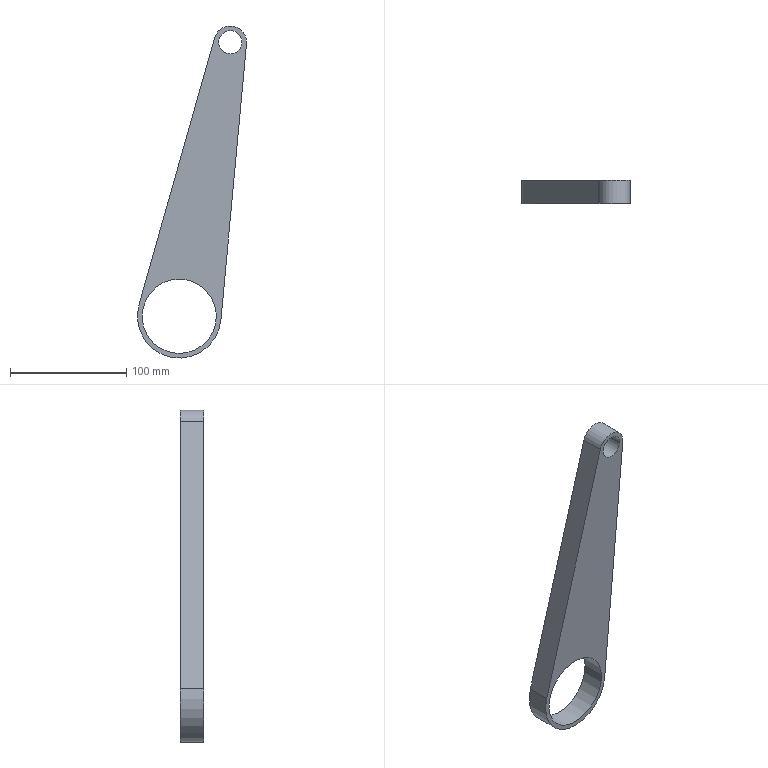Component | NX | CONNECTING_ROD | 1 solid | 8 faces | box 94 x 20 x 285.93 mm | volume 217259 mm3 | plane 4 | cylinder 4 | commonest cylinder face diameters 72 x1 64 x1 28 x1 20 x1
STEP:
#1=CARTESIAN_POINT('',(0.,0.,0.));
#2=DIRECTION('',(0.,0.,1.));
#3=DIRECTION('',(1.,0.,0.));
#4=AXIS2_PLACEMENT_3D('',#1,#2,#3);
#5=CARTESIAN_POINT('',(13.94,312.,234.638));
#6=VERTEX_POINT('',#5);
#7=CARTESIAN_POINT('',(-8.154,312.,-3.328));
#8=VERTEX_POINT('',#7);
#9=CARTESIAN_POINT('',(13.94,312.,234.638));
#10=DIRECTION('',(-0.09245,0.,-0.9957));
#11=VECTOR('',#10,1.);
#12=LINE('',#9,#11);
#13=CARTESIAN_POINT('',(13.94,292.,234.638));
#14=DIRECTION('',(0.9957,0.,-0.09245));
#15=DIRECTION('',(0.09245,0.,0.9957));
#16=AXIS2_PLACEMENT_3D('',#13,#14,#15);
#17=PLANE('',#16);
#18=CARTESIAN_POINT('',(0.,-20.));
#19=DIRECTION('',(-1.,0.));
#20=VECTOR('',#19,1.);
#21=LINE('',#18,#20);
#22=(GEOMETRIC_REPRESENTATION_CONTEXT(2)PARAMETRIC_REPRESENTATION_CONTEXT()REPRESENTATION_CONTEXT('',''));
#23=DEFINITIONAL_REPRESENTATION('',(#21),#22);
#24=PCURVE('',#17,#23);
#25=CARTESIAN_POINT('',(-44.,312.,0.));
#26=DIRECTION('',(0.,1.,0.));
#27=DIRECTION('',(-0.1833,0.,-0.9831));
#28=AXIS2_PLACEMENT_3D('',#25,#26,#27);
#29=PLANE('',#28);
#30=CARTESIAN_POINT('',(-241.283,-13.941));
#31=DIRECTION('',(0.9958,-0.09167));
#32=VECTOR('',#31,1.);
#33=LINE('',#30,#32);
#34=(GEOMETRIC_REPRESENTATION_CONTEXT(2)PARAMETRIC_REPRESENTATION_CONTEXT()REPRESENTATION_CONTEXT('',''));
#35=DEFINITIONAL_REPRESENTATION('',(#33),#34);
#36=PCURVE('',#29,#35);
#37=SURFACE_CURVE('',#12,(#24,#36),.PCURVE_S1.);
#38=EDGE_CURVE('',#6,#8,#37,.T.);
#39=ORIENTED_EDGE('',*,*,#38,.F.);
#40=CARTESIAN_POINT('',(13.94,292.,234.638));
#41=VERTEX_POINT('',#40);
#42=CARTESIAN_POINT('',(13.94,292.,234.638));
#43=DIRECTION('',(0.,1.,0.));
#44=VECTOR('',#43,1.);
#45=LINE('',#42,#44);
#46=CARTESIAN_POINT('',(0.,0.));
#47=DIRECTION('',(0.,-1.));
#48=VECTOR('',#47,1.);
#49=LINE('',#46,#48);
#50=(GEOMETRIC_REPRESENTATION_CONTEXT(2)PARAMETRIC_REPRESENTATION_CONTEXT()REPRESENTATION_CONTEXT('',''));
#51=DEFINITIONAL_REPRESENTATION('',(#49),#50);
#52=PCURVE('',#17,#51);
#53=CARTESIAN_POINT('',(0.,292.,235.932));
#54=DIRECTION('',(0.,1.,0.));
#55=DIRECTION('',(-0.1833,0.,-0.9831));
#56=AXIS2_PLACEMENT_3D('',#53,#54,#55);
#57=CYLINDRICAL_SURFACE('',#56,14.);
#58=CARTESIAN_POINT('',(4.621,0.));
#59=DIRECTION('',(0.,1.));
#60=VECTOR('',#59,1.);
#61=LINE('',#58,#60);
#62=(GEOMETRIC_REPRESENTATION_CONTEXT(2)PARAMETRIC_REPRESENTATION_CONTEXT()REPRESENTATION_CONTEXT('',''));
#63=DEFINITIONAL_REPRESENTATION('',(#61),#62);
#64=PCURVE('',#57,#63);
#65=SURFACE_CURVE('',#45,(#52,#64),.PCURVE_S1.);
#66=EDGE_CURVE('',#41,#6,#65,.T.);
#67=ORIENTED_EDGE('',*,*,#66,.F.);
#68=CARTESIAN_POINT('',(-8.154,292.,-3.328));
#69=VERTEX_POINT('',#68);
#70=CARTESIAN_POINT('',(13.94,292.,234.638));
#71=DIRECTION('',(-0.09245,0.,-0.9957));
#72=VECTOR('',#71,1.);
#73=LINE('',#70,#72);
#74=CARTESIAN_POINT('',(0.,0.));
#75=DIRECTION('',(-1.,0.));
#76=VECTOR('',#75,1.);
#77=LINE('',#74,#76);
#78=(GEOMETRIC_REPRESENTATION_CONTEXT(2)PARAMETRIC_REPRESENTATION_CONTEXT()REPRESENTATION_CONTEXT('',''));
#79=DEFINITIONAL_REPRESENTATION('',(#77),#78);
#80=PCURVE('',#17,#79);
#81=CARTESIAN_POINT('',(-44.,292.,0.));
#82=DIRECTION('',(0.,1.,0.));
#83=DIRECTION('',(-0.1833,0.,-0.9831));
#84=AXIS2_PLACEMENT_3D('',#81,#82,#83);
#85=PLANE('',#84);
#86=CARTESIAN_POINT('',(-241.283,-13.941));
#87=DIRECTION('',(0.9958,-0.09167));
#88=VECTOR('',#87,1.);
#89=LINE('',#86,#88);
#90=(GEOMETRIC_REPRESENTATION_CONTEXT(2)PARAMETRIC_REPRESENTATION_CONTEXT()REPRESENTATION_CONTEXT('',''));
#91=DEFINITIONAL_REPRESENTATION('',(#89),#90);
#92=PCURVE('',#85,#91);
#93=SURFACE_CURVE('',#73,(#80,#92),.PCURVE_S1.);
#94=EDGE_CURVE('',#41,#69,#93,.T.);
#95=ORIENTED_EDGE('',*,*,#94,.T.);
#96=CARTESIAN_POINT('',(-8.154,292.,-3.328));
#97=DIRECTION('',(0.,1.,0.));
#98=VECTOR('',#97,1.);
#99=LINE('',#96,#98);
#100=CARTESIAN_POINT('',(-238.99,0.));
#101=DIRECTION('',(0.,-1.));
#102=VECTOR('',#101,1.);
#103=LINE('',#100,#102);
#104=(GEOMETRIC_REPRESENTATION_CONTEXT(2)PARAMETRIC_REPRESENTATION_CONTEXT()REPRESENTATION_CONTEXT('',''));
#105=DEFINITIONAL_REPRESENTATION('',(#103),#104);
#106=PCURVE('',#17,#105);
#107=CARTESIAN_POINT('',(-44.,292.,0.));
#108=DIRECTION('',(0.,1.,0.));
#109=DIRECTION('',(-0.1833,0.,-0.9831));
#110=AXIS2_PLACEMENT_3D('',#107,#108,#109);
#111=CYLINDRICAL_SURFACE('',#110,36.);
#112=CARTESIAN_POINT('',(4.621,0.));
#113=DIRECTION('',(0.,1.));
#114=VECTOR('',#113,1.);
#115=LINE('',#112,#114);
#116=(GEOMETRIC_REPRESENTATION_CONTEXT(2)PARAMETRIC_REPRESENTATION_CONTEXT()REPRESENTATION_CONTEXT('',''));
#117=DEFINITIONAL_REPRESENTATION('',(#115),#116);
#118=PCURVE('',#111,#117);
#119=SURFACE_CURVE('',#99,(#106,#118),.PCURVE_S1.);
#120=EDGE_CURVE('',#69,#8,#119,.T.);
#121=ORIENTED_EDGE('',*,*,#120,.T.);
#122=EDGE_LOOP('',(#39,#67,#95,#121));
#123=FACE_BOUND('',#122,.T.);
#124=ADVANCED_FACE('',(#123),#17,.T.);
#125=CARTESIAN_POINT('',(-78.636,312.,9.816));
#126=VERTEX_POINT('',#125);
#127=CARTESIAN_POINT('',(-44.,312.,0.));
#128=DIRECTION('',(0.,1.,0.));
#129=DIRECTION('',(-0.9831,0.,0.1833));
#130=AXIS2_PLACEMENT_3D('',#127,#128,#129);
#131=CIRCLE('',#130,36.);
#132=CARTESIAN_POINT('',(1.571,20.));
#133=DIRECTION('',(1.,0.));
#134=VECTOR('',#133,1.);
#135=LINE('',#132,#134);
#136=(GEOMETRIC_REPRESENTATION_CONTEXT(2)PARAMETRIC_REPRESENTATION_CONTEXT()REPRESENTATION_CONTEXT('',''));
#137=DEFINITIONAL_REPRESENTATION('',(#135),#136);
#138=PCURVE('',#111,#137);
#139=CARTESIAN_POINT('',(0.,0.));
#140=DIRECTION('',(0.,1.));
#141=AXIS2_PLACEMENT_2D('',#139,#140);
#142=CIRCLE('',#141,36.);
#143=(GEOMETRIC_REPRESENTATION_CONTEXT(2)PARAMETRIC_REPRESENTATION_CONTEXT()REPRESENTATION_CONTEXT('',''));
#144=DEFINITIONAL_REPRESENTATION('',(#142),#143);
#145=PCURVE('',#29,#144);
#146=SURFACE_CURVE('',#131,(#138,#145),.PCURVE_S1.);
#147=EDGE_CURVE('',#8,#126,#146,.T.);
#148=ORIENTED_EDGE('',*,*,#147,.F.);
#149=ORIENTED_EDGE('',*,*,#120,.F.);
#150=CARTESIAN_POINT('',(-78.636,292.,9.816));
#151=VERTEX_POINT('',#150);
#152=CARTESIAN_POINT('',(-44.,292.,0.));
#153=DIRECTION('',(0.,1.,0.));
#154=DIRECTION('',(-0.9831,0.,0.1833));
#155=AXIS2_PLACEMENT_3D('',#152,#153,#154);
#156=CIRCLE('',#155,36.);
#157=CARTESIAN_POINT('',(1.571,0.));
#158=DIRECTION('',(1.,0.));
#159=VECTOR('',#158,1.);
#160=LINE('',#157,#159);
#161=(GEOMETRIC_REPRESENTATION_CONTEXT(2)PARAMETRIC_REPRESENTATION_CONTEXT()REPRESENTATION_CONTEXT('',''));
#162=DEFINITIONAL_REPRESENTATION('',(#160),#161);
#163=PCURVE('',#111,#162);
#164=CARTESIAN_POINT('',(0.,0.));
#165=DIRECTION('',(0.,1.));
#166=AXIS2_PLACEMENT_2D('',#164,#165);
#167=CIRCLE('',#166,36.);
#168=(GEOMETRIC_REPRESENTATION_CONTEXT(2)PARAMETRIC_REPRESENTATION_CONTEXT()REPRESENTATION_CONTEXT('',''));
#169=DEFINITIONAL_REPRESENTATION('',(#167),#168);
#170=PCURVE('',#85,#169);
#171=SURFACE_CURVE('',#156,(#163,#170),.PCURVE_S1.);
#172=EDGE_CURVE('',#69,#151,#171,.T.);
#173=ORIENTED_EDGE('',*,*,#172,.T.);
#174=CARTESIAN_POINT('',(-78.636,292.,9.816));
#175=DIRECTION('',(0.,1.,0.));
#176=VECTOR('',#175,1.);
#177=LINE('',#174,#176);
#178=CARTESIAN_POINT('',(7.946,0.));
#179=DIRECTION('',(0.,1.));
#180=VECTOR('',#179,1.);
#181=LINE('',#178,#180);
#182=(GEOMETRIC_REPRESENTATION_CONTEXT(2)PARAMETRIC_REPRESENTATION_CONTEXT()REPRESENTATION_CONTEXT('',''));
#183=DEFINITIONAL_REPRESENTATION('',(#181),#182);
#184=PCURVE('',#111,#183);
#185=CARTESIAN_POINT('',(-78.636,292.,9.816));
#186=DIRECTION('',(-0.9621,0.,0.2727));
#187=DIRECTION('',(-0.2727,0.,-0.9621));
#188=AXIS2_PLACEMENT_3D('',#185,#186,#187);
#189=PLANE('',#188);
#190=CARTESIAN_POINT('',(0.,0.));
#191=DIRECTION('',(0.,-1.));
#192=VECTOR('',#191,1.);
#193=LINE('',#190,#192);
#194=(GEOMETRIC_REPRESENTATION_CONTEXT(2)PARAMETRIC_REPRESENTATION_CONTEXT()REPRESENTATION_CONTEXT('',''));
#195=DEFINITIONAL_REPRESENTATION('',(#193),#194);
#196=PCURVE('',#189,#195);
#197=SURFACE_CURVE('',#177,(#184,#196),.PCURVE_S1.);
#198=EDGE_CURVE('',#151,#126,#197,.T.);
#199=ORIENTED_EDGE('',*,*,#198,.T.);
#200=EDGE_LOOP('',(#148,#149,#173,#199));
#201=FACE_BOUND('',#200,.T.);
#202=ADVANCED_FACE('',(#201),#111,.T.);
#203=CARTESIAN_POINT('',(-13.469,312.,239.75));
#204=VERTEX_POINT('',#203);
#205=CARTESIAN_POINT('',(-78.636,312.,9.816));
#206=DIRECTION('',(0.2727,0.,0.9621));
#207=VECTOR('',#206,1.);
#208=LINE('',#205,#207);
#209=CARTESIAN_POINT('',(0.,-20.));
#210=DIRECTION('',(-1.,0.));
#211=VECTOR('',#210,1.);
#212=LINE('',#209,#211);
#213=(GEOMETRIC_REPRESENTATION_CONTEXT(2)PARAMETRIC_REPRESENTATION_CONTEXT()REPRESENTATION_CONTEXT('',''));
#214=DEFINITIONAL_REPRESENTATION('',(#212),#213);
#215=PCURVE('',#189,#214);
#216=CARTESIAN_POINT('',(-3.3,35.848));
#217=DIRECTION('',(-0.9958,-0.09167));
#218=VECTOR('',#217,1.);
#219=LINE('',#216,#218);
#220=(GEOMETRIC_REPRESENTATION_CONTEXT(2)PARAMETRIC_REPRESENTATION_CONTEXT()REPRESENTATION_CONTEXT('',''));
#221=DEFINITIONAL_REPRESENTATION('',(#219),#220);
#222=PCURVE('',#29,#221);
#223=SURFACE_CURVE('',#208,(#215,#222),.PCURVE_S1.);
#224=EDGE_CURVE('',#126,#204,#223,.T.);
#225=ORIENTED_EDGE('',*,*,#224,.F.);
#226=ORIENTED_EDGE('',*,*,#198,.F.);
#227=CARTESIAN_POINT('',(-13.469,292.,239.75));
#228=VERTEX_POINT('',#227);
#229=CARTESIAN_POINT('',(-78.636,292.,9.816));
#230=DIRECTION('',(0.2727,0.,0.9621));
#231=VECTOR('',#230,1.);
#232=LINE('',#229,#231);
#233=CARTESIAN_POINT('',(0.,0.));
#234=DIRECTION('',(-1.,0.));
#235=VECTOR('',#234,1.);
#236=LINE('',#233,#235);
#237=(GEOMETRIC_REPRESENTATION_CONTEXT(2)PARAMETRIC_REPRESENTATION_CONTEXT()REPRESENTATION_CONTEXT('',''));
#238=DEFINITIONAL_REPRESENTATION('',(#236),#237);
#239=PCURVE('',#189,#238);
#240=CARTESIAN_POINT('',(-3.3,35.848));
#241=DIRECTION('',(-0.9958,-0.09167));
#242=VECTOR('',#241,1.);
#243=LINE('',#240,#242);
#244=(GEOMETRIC_REPRESENTATION_CONTEXT(2)PARAMETRIC_REPRESENTATION_CONTEXT()REPRESENTATION_CONTEXT('',''));
#245=DEFINITIONAL_REPRESENTATION('',(#243),#244);
#246=PCURVE('',#85,#245);
#247=SURFACE_CURVE('',#232,(#239,#246),.PCURVE_S1.);
#248=EDGE_CURVE('',#151,#228,#247,.T.);
#249=ORIENTED_EDGE('',*,*,#248,.T.);
#250=CARTESIAN_POINT('',(-13.469,292.,239.75));
#251=DIRECTION('',(0.,1.,0.));
#252=VECTOR('',#251,1.);
#253=LINE('',#250,#252);
#254=CARTESIAN_POINT('',(-238.99,0.));
#255=DIRECTION('',(0.,-1.));
#256=VECTOR('',#255,1.);
#257=LINE('',#254,#256);
#258=(GEOMETRIC_REPRESENTATION_CONTEXT(2)PARAMETRIC_REPRESENTATION_CONTEXT()REPRESENTATION_CONTEXT('',''));
#259=DEFINITIONAL_REPRESENTATION('',(#257),#258);
#260=PCURVE('',#189,#259);
#261=CARTESIAN_POINT('',(1.663,0.));
#262=DIRECTION('',(0.,1.));
#263=VECTOR('',#262,1.);
#264=LINE('',#261,#263);
#265=(GEOMETRIC_REPRESENTATION_CONTEXT(2)PARAMETRIC_REPRESENTATION_CONTEXT()REPRESENTATION_CONTEXT('',''));
#266=DEFINITIONAL_REPRESENTATION('',(#264),#265);
#267=PCURVE('',#57,#266);
#268=SURFACE_CURVE('',#253,(#260,#267),.PCURVE_S1.);
#269=EDGE_CURVE('',#228,#204,#268,.T.);
#270=ORIENTED_EDGE('',*,*,#269,.T.);
#271=EDGE_LOOP('',(#225,#226,#249,#270));
#272=FACE_BOUND('',#271,.T.);
#273=ADVANCED_FACE('',(#272),#189,.T.);
#274=CARTESIAN_POINT('',(-75.458,292.,5.867));
#275=VERTEX_POINT('',#274);
#276=CARTESIAN_POINT('',(-44.,292.,0.));
#277=DIRECTION('',(0.,1.,0.));
#278=DIRECTION('',(-0.9831,0.,0.1833));
#279=AXIS2_PLACEMENT_3D('',#276,#277,#278);
#280=CIRCLE('',#279,32.);
#281=CARTESIAN_POINT('',(-44.,292.,0.));
#282=DIRECTION('',(0.,1.,0.));
#283=DIRECTION('',(-0.1833,0.,-0.9831));
#284=AXIS2_PLACEMENT_3D('',#281,#282,#283);
#285=CYLINDRICAL_SURFACE('',#284,32.);
#286=CARTESIAN_POINT('',(1.571,0.));
#287=DIRECTION('',(1.,0.));
#288=VECTOR('',#287,1.);
#289=LINE('',#286,#288);
#290=(GEOMETRIC_REPRESENTATION_CONTEXT(2)PARAMETRIC_REPRESENTATION_CONTEXT()REPRESENTATION_CONTEXT('',''));
#291=DEFINITIONAL_REPRESENTATION('',(#289),#290);
#292=PCURVE('',#285,#291);
#293=CARTESIAN_POINT('',(0.,0.));
#294=DIRECTION('',(0.,1.));
#295=AXIS2_PLACEMENT_2D('',#293,#294);
#296=CIRCLE('',#295,32.);
#297=(GEOMETRIC_REPRESENTATION_CONTEXT(2)PARAMETRIC_REPRESENTATION_CONTEXT()REPRESENTATION_CONTEXT('',''));
#298=DEFINITIONAL_REPRESENTATION('',(#296),#297);
#299=PCURVE('',#85,#298);
#300=SURFACE_CURVE('',#280,(#292,#299),.PCURVE_S1.);
#301=EDGE_CURVE('',#275,#275,#300,.T.);
#302=ORIENTED_EDGE('',*,*,#301,.T.);
#303=CARTESIAN_POINT('',(-75.458,312.,5.867));
#304=VERTEX_POINT('',#303);
#305=CARTESIAN_POINT('',(-75.458,292.,5.867));
#306=CARTESIAN_POINT('',(-75.458,312.,5.867));
#307=B_SPLINE_CURVE_WITH_KNOTS('',1,(#305,#306),.UNSPECIFIED.,.F.,.F.,(2,2),(0.,20.),.PIECEWISE_BEZIER_KNOTS.);
#308=CARTESIAN_POINT('',(7.854,0.));
#309=DIRECTION('',(0.,1.));
#310=VECTOR('',#309,1.);
#311=LINE('',#308,#310);
#312=(GEOMETRIC_REPRESENTATION_CONTEXT(2)PARAMETRIC_REPRESENTATION_CONTEXT()REPRESENTATION_CONTEXT('',''));
#313=DEFINITIONAL_REPRESENTATION('',(#311),#312);
#314=PCURVE('',#285,#313);
#315=CARTESIAN_POINT('',(1.571,0.));
#316=DIRECTION('',(0.,1.));
#317=VECTOR('',#316,1.);
#318=LINE('',#315,#317);
#319=(GEOMETRIC_REPRESENTATION_CONTEXT(2)PARAMETRIC_REPRESENTATION_CONTEXT()REPRESENTATION_CONTEXT('',''));
#320=DEFINITIONAL_REPRESENTATION('',(#318),#319);
#321=PCURVE('',#285,#320);
#322=SEAM_CURVE('',#307,(#314,#321),.PCURVE_S1.);
#323=EDGE_CURVE('',#275,#304,#322,.T.);
#324=ORIENTED_EDGE('',*,*,#323,.T.);
#325=CARTESIAN_POINT('',(-44.,312.,0.));
#326=DIRECTION('',(0.,1.,0.));
#327=DIRECTION('',(-0.9831,0.,0.1833));
#328=AXIS2_PLACEMENT_3D('',#325,#326,#327);
#329=CIRCLE('',#328,32.);
#330=CARTESIAN_POINT('',(1.571,20.));
#331=DIRECTION('',(1.,0.));
#332=VECTOR('',#331,1.);
#333=LINE('',#330,#332);
#334=(GEOMETRIC_REPRESENTATION_CONTEXT(2)PARAMETRIC_REPRESENTATION_CONTEXT()REPRESENTATION_CONTEXT('',''));
#335=DEFINITIONAL_REPRESENTATION('',(#333),#334);
#336=PCURVE('',#285,#335);
#337=CARTESIAN_POINT('',(0.,0.));
#338=DIRECTION('',(0.,1.));
#339=AXIS2_PLACEMENT_2D('',#337,#338);
#340=CIRCLE('',#339,32.);
#341=(GEOMETRIC_REPRESENTATION_CONTEXT(2)PARAMETRIC_REPRESENTATION_CONTEXT()REPRESENTATION_CONTEXT('',''));
#342=DEFINITIONAL_REPRESENTATION('',(#340),#341);
#343=PCURVE('',#29,#342);
#344=SURFACE_CURVE('',#329,(#336,#343),.PCURVE_S1.);
#345=EDGE_CURVE('',#304,#304,#344,.T.);
#346=ORIENTED_EDGE('',*,*,#345,.F.);
#347=ORIENTED_EDGE('',*,*,#323,.F.);
#348=EDGE_LOOP('',(#302,#324,#346,#347));
#349=FACE_BOUND('',#348,.F.);
#350=ADVANCED_FACE('',(#349),#285,.F.);
#351=CARTESIAN_POINT('',(0.,312.,235.932));
#352=DIRECTION('',(0.,1.,0.));
#353=DIRECTION('',(-0.9831,0.,0.1833));
#354=AXIS2_PLACEMENT_3D('',#351,#352,#353);
#355=CIRCLE('',#354,14.);
#356=CARTESIAN_POINT('',(1.571,20.));
#357=DIRECTION('',(1.,0.));
#358=VECTOR('',#357,1.);
#359=LINE('',#356,#358);
#360=(GEOMETRIC_REPRESENTATION_CONTEXT(2)PARAMETRIC_REPRESENTATION_CONTEXT()REPRESENTATION_CONTEXT('',''));
#361=DEFINITIONAL_REPRESENTATION('',(#359),#360);
#362=PCURVE('',#57,#361);
#363=CARTESIAN_POINT('',(-240.,0.));
#364=DIRECTION('',(0.,1.));
#365=AXIS2_PLACEMENT_2D('',#363,#364);
#366=CIRCLE('',#365,14.);
#367=(GEOMETRIC_REPRESENTATION_CONTEXT(2)PARAMETRIC_REPRESENTATION_CONTEXT()REPRESENTATION_CONTEXT('',''));
#368=DEFINITIONAL_REPRESENTATION('',(#366),#367);
#369=PCURVE('',#29,#368);
#370=SURFACE_CURVE('',#355,(#362,#369),.PCURVE_S1.);
#371=EDGE_CURVE('',#204,#6,#370,.T.);
#372=ORIENTED_EDGE('',*,*,#371,.F.);
#373=ORIENTED_EDGE('',*,*,#269,.F.);
#374=CARTESIAN_POINT('',(0.,292.,235.932));
#375=DIRECTION('',(0.,1.,0.));
#376=DIRECTION('',(-0.9831,0.,0.1833));
#377=AXIS2_PLACEMENT_3D('',#374,#375,#376);
#378=CIRCLE('',#377,14.);
#379=CARTESIAN_POINT('',(1.571,0.));
#380=DIRECTION('',(1.,0.));
#381=VECTOR('',#380,1.);
#382=LINE('',#379,#381);
#383=(GEOMETRIC_REPRESENTATION_CONTEXT(2)PARAMETRIC_REPRESENTATION_CONTEXT()REPRESENTATION_CONTEXT('',''));
#384=DEFINITIONAL_REPRESENTATION('',(#382),#383);
#385=PCURVE('',#57,#384);
#386=CARTESIAN_POINT('',(-240.,0.));
#387=DIRECTION('',(0.,1.));
#388=AXIS2_PLACEMENT_2D('',#386,#387);
#389=CIRCLE('',#388,14.);
#390=(GEOMETRIC_REPRESENTATION_CONTEXT(2)PARAMETRIC_REPRESENTATION_CONTEXT()REPRESENTATION_CONTEXT('',''));
#391=DEFINITIONAL_REPRESENTATION('',(#389),#390);
#392=PCURVE('',#85,#391);
#393=SURFACE_CURVE('',#378,(#385,#392),.PCURVE_S1.);
#394=EDGE_CURVE('',#228,#41,#393,.T.);
#395=ORIENTED_EDGE('',*,*,#394,.T.);
#396=ORIENTED_EDGE('',*,*,#66,.T.);
#397=EDGE_LOOP('',(#372,#373,#395,#396));
#398=FACE_BOUND('',#397,.T.);
#399=ADVANCED_FACE('',(#398),#57,.T.);
#400=CARTESIAN_POINT('',(-9.831,292.,237.766));
#401=VERTEX_POINT('',#400);
#402=CARTESIAN_POINT('',(0.,292.,235.932));
#403=DIRECTION('',(0.,1.,0.));
#404=DIRECTION('',(-0.9831,0.,0.1833));
#405=AXIS2_PLACEMENT_3D('',#402,#403,#404);
#406=CIRCLE('',#405,10.);
#407=CARTESIAN_POINT('',(0.,292.,235.932));
#408=DIRECTION('',(0.,1.,0.));
#409=DIRECTION('',(-0.1833,0.,-0.9831));
#410=AXIS2_PLACEMENT_3D('',#407,#408,#409);
#411=CYLINDRICAL_SURFACE('',#410,10.);
#412=CARTESIAN_POINT('',(1.571,0.));
#413=DIRECTION('',(1.,0.));
#414=VECTOR('',#413,1.);
#415=LINE('',#412,#414);
#416=(GEOMETRIC_REPRESENTATION_CONTEXT(2)PARAMETRIC_REPRESENTATION_CONTEXT()REPRESENTATION_CONTEXT('',''));
#417=DEFINITIONAL_REPRESENTATION('',(#415),#416);
#418=PCURVE('',#411,#417);
#419=CARTESIAN_POINT('',(-240.,0.));
#420=DIRECTION('',(0.,1.));
#421=AXIS2_PLACEMENT_2D('',#419,#420);
#422=CIRCLE('',#421,10.);
#423=(GEOMETRIC_REPRESENTATION_CONTEXT(2)PARAMETRIC_REPRESENTATION_CONTEXT()REPRESENTATION_CONTEXT('',''));
#424=DEFINITIONAL_REPRESENTATION('',(#422),#423);
#425=PCURVE('',#85,#424);
#426=SURFACE_CURVE('',#406,(#418,#425),.PCURVE_S1.);
#427=EDGE_CURVE('',#401,#401,#426,.T.);
#428=ORIENTED_EDGE('',*,*,#427,.T.);
#429=CARTESIAN_POINT('',(-9.831,312.,237.766));
#430=VERTEX_POINT('',#429);
#431=CARTESIAN_POINT('',(-9.831,292.,237.766));
#432=CARTESIAN_POINT('',(-9.831,312.,237.766));
#433=B_SPLINE_CURVE_WITH_KNOTS('',1,(#431,#432),.UNSPECIFIED.,.F.,.F.,(2,2),(0.,20.),.PIECEWISE_BEZIER_KNOTS.);
#434=CARTESIAN_POINT('',(7.854,0.));
#435=DIRECTION('',(0.,1.));
#436=VECTOR('',#435,1.);
#437=LINE('',#434,#436);
#438=(GEOMETRIC_REPRESENTATION_CONTEXT(2)PARAMETRIC_REPRESENTATION_CONTEXT()REPRESENTATION_CONTEXT('',''));
#439=DEFINITIONAL_REPRESENTATION('',(#437),#438);
#440=PCURVE('',#411,#439);
#441=CARTESIAN_POINT('',(1.571,0.));
#442=DIRECTION('',(0.,1.));
#443=VECTOR('',#442,1.);
#444=LINE('',#441,#443);
#445=(GEOMETRIC_REPRESENTATION_CONTEXT(2)PARAMETRIC_REPRESENTATION_CONTEXT()REPRESENTATION_CONTEXT('',''));
#446=DEFINITIONAL_REPRESENTATION('',(#444),#445);
#447=PCURVE('',#411,#446);
#448=SEAM_CURVE('',#433,(#440,#447),.PCURVE_S1.);
#449=EDGE_CURVE('',#401,#430,#448,.T.);
#450=ORIENTED_EDGE('',*,*,#449,.T.);
#451=CARTESIAN_POINT('',(0.,312.,235.932));
#452=DIRECTION('',(0.,1.,0.));
#453=DIRECTION('',(-0.9831,0.,0.1833));
#454=AXIS2_PLACEMENT_3D('',#451,#452,#453);
#455=CIRCLE('',#454,10.);
#456=CARTESIAN_POINT('',(1.571,20.));
#457=DIRECTION('',(1.,0.));
#458=VECTOR('',#457,1.);
#459=LINE('',#456,#458);
#460=(GEOMETRIC_REPRESENTATION_CONTEXT(2)PARAMETRIC_REPRESENTATION_CONTEXT()REPRESENTATION_CONTEXT('',''));
#461=DEFINITIONAL_REPRESENTATION('',(#459),#460);
#462=PCURVE('',#411,#461);
#463=CARTESIAN_POINT('',(-240.,0.));
#464=DIRECTION('',(0.,1.));
#465=AXIS2_PLACEMENT_2D('',#463,#464);
#466=CIRCLE('',#465,10.);
#467=(GEOMETRIC_REPRESENTATION_CONTEXT(2)PARAMETRIC_REPRESENTATION_CONTEXT()REPRESENTATION_CONTEXT('',''));
#468=DEFINITIONAL_REPRESENTATION('',(#466),#467);
#469=PCURVE('',#29,#468);
#470=SURFACE_CURVE('',#455,(#462,#469),.PCURVE_S1.);
#471=EDGE_CURVE('',#430,#430,#470,.T.);
#472=ORIENTED_EDGE('',*,*,#471,.F.);
#473=ORIENTED_EDGE('',*,*,#449,.F.);
#474=EDGE_LOOP('',(#428,#450,#472,#473));
#475=FACE_BOUND('',#474,.F.);
#476=ADVANCED_FACE('',(#475),#411,.F.);
#477=ORIENTED_EDGE('',*,*,#94,.F.);
#478=ORIENTED_EDGE('',*,*,#394,.F.);
#479=ORIENTED_EDGE('',*,*,#248,.F.);
#480=ORIENTED_EDGE('',*,*,#172,.F.);
#481=EDGE_LOOP('',(#477,#478,#479,#480));
#482=FACE_BOUND('',#481,.T.);
#483=ORIENTED_EDGE('',*,*,#301,.T.);
#484=EDGE_LOOP('',(#483));
#485=FACE_BOUND('',#484,.T.);
#486=ORIENTED_EDGE('',*,*,#427,.T.);
#487=EDGE_LOOP('',(#486));
#488=FACE_BOUND('',#487,.T.);
#489=ADVANCED_FACE('',(#482,#485,#488),#85,.F.);
#490=ORIENTED_EDGE('',*,*,#38,.T.);
#491=ORIENTED_EDGE('',*,*,#147,.T.);
#492=ORIENTED_EDGE('',*,*,#224,.T.);
#493=ORIENTED_EDGE('',*,*,#371,.T.);
#494=EDGE_LOOP('',(#490,#491,#492,#493));
#495=FACE_BOUND('',#494,.T.);
#496=ORIENTED_EDGE('',*,*,#345,.F.);
#497=EDGE_LOOP('',(#496));
#498=FACE_BOUND('',#497,.T.);
#499=ORIENTED_EDGE('',*,*,#471,.F.);
#500=EDGE_LOOP('',(#499));
#501=FACE_BOUND('',#500,.T.);
#502=ADVANCED_FACE('',(#495,#498,#501),#29,.T.);
#503=CLOSED_SHELL('',(#124,#202,#273,#350,#399,#476,#489,#502));
#504=MANIFOLD_SOLID_BREP('',#503);
#505=(LENGTH_UNIT()NAMED_UNIT(*)SI_UNIT(.MILLI.,.METRE.));
#506=UNCERTAINTY_MEASURE_WITH_UNIT(LENGTH_MEASURE(0.000002),#505,'','');
#507=(NAMED_UNIT(*)PLANE_ANGLE_UNIT()SI_UNIT($,.RADIAN.));
#508=(NAMED_UNIT(*)SI_UNIT($,.STERADIAN.)SOLID_ANGLE_UNIT());
#509=(GEOMETRIC_REPRESENTATION_CONTEXT(3)GLOBAL_UNCERTAINTY_ASSIGNED_CONTEXT((#506))GLOBAL_UNIT_ASSIGNED_CONTEXT((#505,#507,#508))REPRESENTATION_CONTEXT('',''));
#510=ADVANCED_BREP_SHAPE_REPRESENTATION('',(#4,#504),#509);